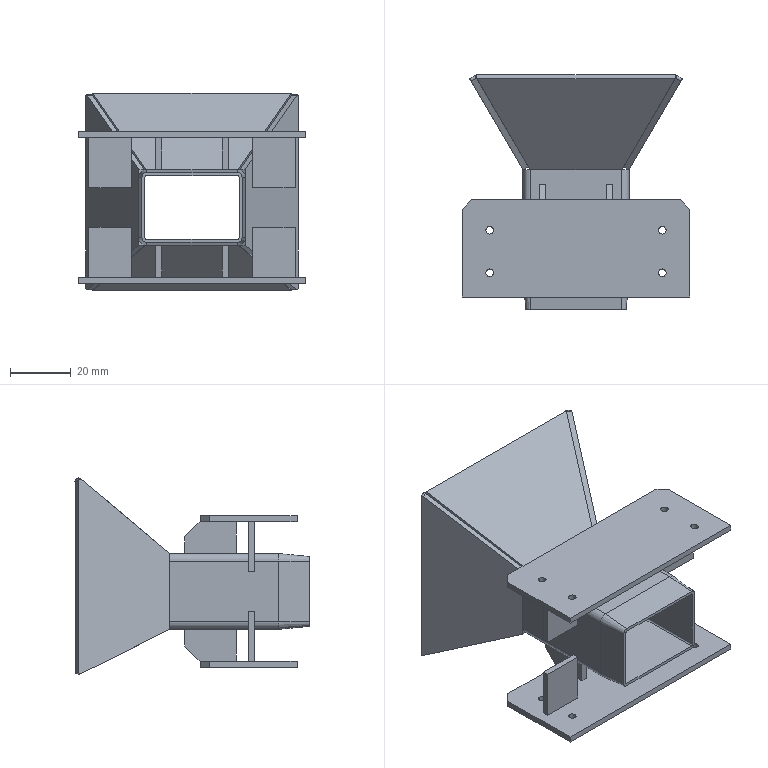Component | SolidWorks | BAssemblyInnerBagFunnel-1_InnerBagFunnel1-1 | 15 solids | 140 faces | volume 35380 mm3 | plane 108 | cylinder 28 | cone 4 | commonest cylinder face diameters 2.5 x16 5 x4 1 x4 1.2 x4